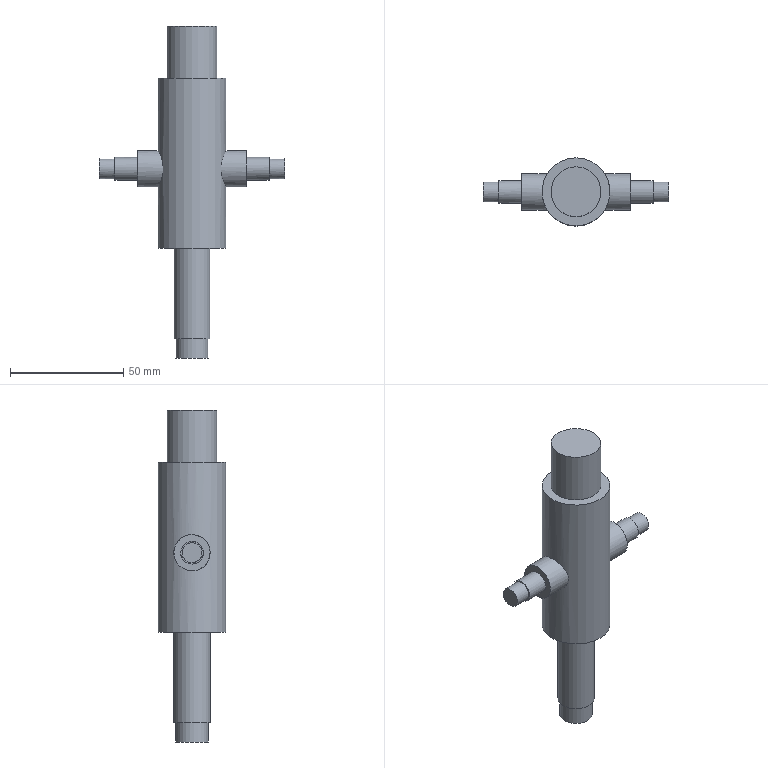Component | NX | 2 | 1 solid | 21 faces | volume 77443 mm3 | plane 11 | cylinder 10 | commonest cylinder face diameters 16 x3 10 x2 8.782 x2 30 x1 22 x1 14.376 x1